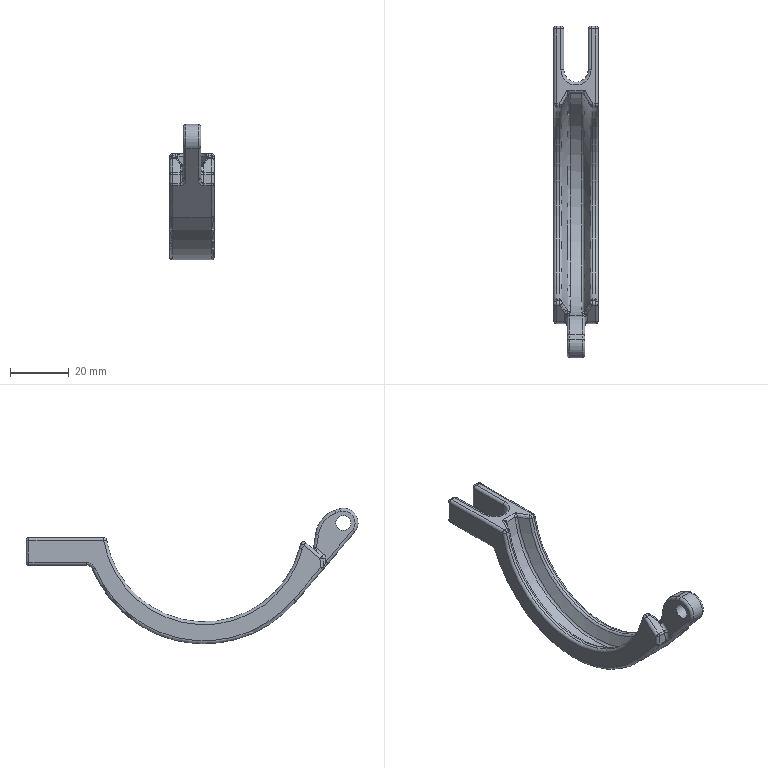Component | NX | BOTTOM_BUCKLE | 1 solid | 137 faces | volume 11219 mm3 | cylinder 49 | spline 27 | torus 24 | sphere 20 | plane 15 | cone 2 | commonest cylinder face diameters 2 x37 38.209 x3 67.5 x2 82.5 x1 10 x1 8.3 x1 4 x1 76.5 x1